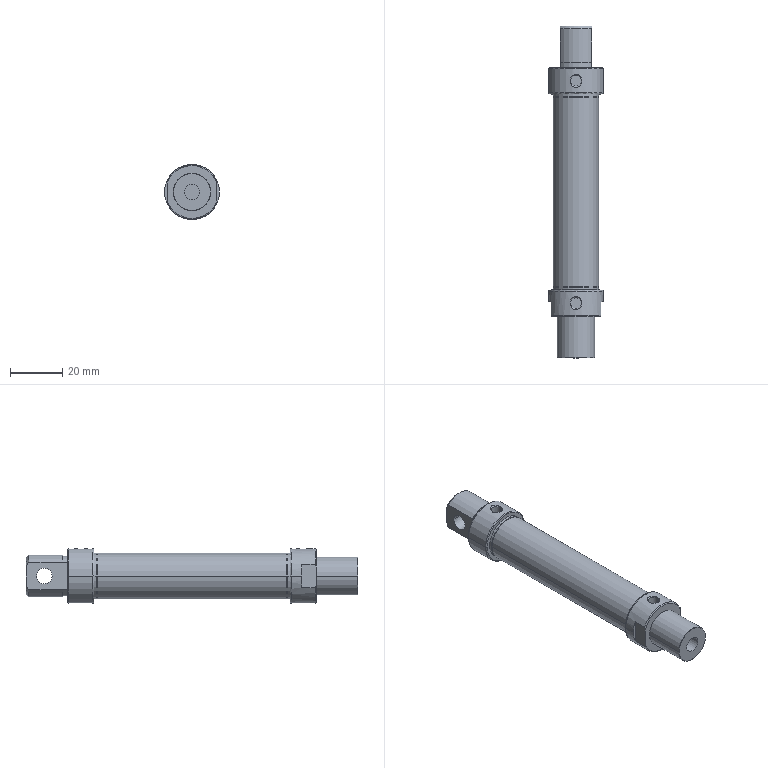Component | SolidWorks | gbgbMA16x35SCA_0_+-2_gbgb1-1 | 1 solid | 66 faces | volume 17409 mm3 | cylinder 26 | plane 20 | cone 12 | spline 8 | commonest cylinder face diameters 17.4 x6 21 x4 4.134 x4 6 x4 16 x4 14.376 x2 15.7 x2